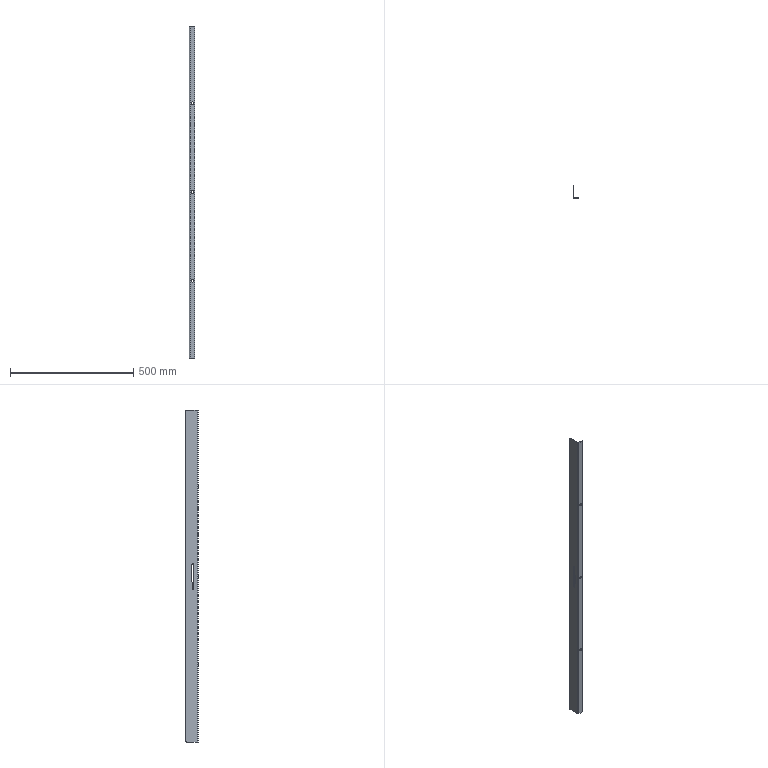Component | SolidWorks | RearRightSidePlateAssembly-1_RearRightSidePanelVerticalRib1-1 | 1 solid | 29 faces | box 24 x 50 x 1345 mm | volume 188474 mm3 | plane 18 | cylinder 11 | commonest cylinder face diameters 10 x6 6 x3 8 x1 4 x1 | material Plain Carbon Steel
STEP:
#1=CARTESIAN_POINT('',(78.003,47.699,67.145));
#2=VERTEX_POINT('',#1);
#3=CARTESIAN_POINT('',(78.003,47.699,67.539));
#4=VERTEX_POINT('',#3);
#5=CARTESIAN_POINT('',(78.003,47.699,67.342));
#6=DIRECTION('',(-0.,1.,0.));
#7=DIRECTION('',(0.,0.,1.));
#8=AXIS2_PLACEMENT_3D('',#5,#6,#7);
#9=CIRCLE('',#8,0.1969);
#10=EDGE_CURVE('',#2,#4,#9,.T.);
#11=ORIENTED_EDGE('',*,*,#10,.F.);
#12=CARTESIAN_POINT('',(78.003,47.778,67.145));
#13=VERTEX_POINT('',#12);
#14=CARTESIAN_POINT('',(78.003,47.699,67.145));
#15=DIRECTION('',(-0.,1.,0.));
#16=VECTOR('',#15,39.37);
#17=LINE('',#14,#16);
#18=EDGE_CURVE('',#2,#13,#17,.T.);
#19=ORIENTED_EDGE('',*,*,#18,.T.);
#20=CARTESIAN_POINT('',(78.003,47.778,67.539));
#21=VERTEX_POINT('',#20);
#22=CARTESIAN_POINT('',(78.003,47.778,67.342));
#23=DIRECTION('',(-0.,1.,0.));
#24=DIRECTION('',(0.,0.,1.));
#25=AXIS2_PLACEMENT_3D('',#22,#23,#24);
#26=CIRCLE('',#25,0.1969);
#27=EDGE_CURVE('',#13,#21,#26,.T.);
#28=ORIENTED_EDGE('',*,*,#27,.T.);
#29=CARTESIAN_POINT('',(78.003,47.699,67.539));
#30=DIRECTION('',(-0.,1.,0.));
#31=VECTOR('',#30,39.37);
#32=LINE('',#29,#31);
#33=EDGE_CURVE('',#4,#21,#32,.T.);
#34=ORIENTED_EDGE('',*,*,#33,.F.);
#35=EDGE_LOOP('',(#11,#19,#28,#34));
#36=FACE_OUTER_BOUND('',#35,.T.);
#37=CARTESIAN_POINT('',(78.003,47.699,67.342));
#38=DIRECTION('',(-0.,1.,0.));
#39=DIRECTION('',(0.,0.,1.));
#40=AXIS2_PLACEMENT_3D('',#37,#38,#39);
#41=CYLINDRICAL_SURFACE('',#40,0.1969);
#42=ADVANCED_FACE('',(#36),#41,.F.);
#43=CARTESIAN_POINT('',(78.003,47.699,38.798));
#44=VERTEX_POINT('',#43);
#45=CARTESIAN_POINT('',(78.003,47.699,39.192));
#46=VERTEX_POINT('',#45);
#47=CARTESIAN_POINT('',(78.003,47.699,38.995));
#48=DIRECTION('',(-0.,1.,0.));
#49=DIRECTION('',(0.,0.,1.));
#50=AXIS2_PLACEMENT_3D('',#47,#48,#49);
#51=CIRCLE('',#50,0.1969);
#52=EDGE_CURVE('',#44,#46,#51,.T.);
#53=ORIENTED_EDGE('',*,*,#52,.F.);
#54=CARTESIAN_POINT('',(78.003,47.778,38.798));
#55=VERTEX_POINT('',#54);
#56=CARTESIAN_POINT('',(78.003,47.699,38.798));
#57=DIRECTION('',(-0.,1.,0.));
#58=VECTOR('',#57,39.37);
#59=LINE('',#56,#58);
#60=EDGE_CURVE('',#44,#55,#59,.T.);
#61=ORIENTED_EDGE('',*,*,#60,.T.);
#62=CARTESIAN_POINT('',(78.003,47.778,39.192));
#63=VERTEX_POINT('',#62);
#64=CARTESIAN_POINT('',(78.003,47.778,38.995));
#65=DIRECTION('',(-0.,1.,0.));
#66=DIRECTION('',(0.,0.,1.));
#67=AXIS2_PLACEMENT_3D('',#64,#65,#66);
#68=CIRCLE('',#67,0.1969);
#69=EDGE_CURVE('',#55,#63,#68,.T.);
#70=ORIENTED_EDGE('',*,*,#69,.T.);
#71=CARTESIAN_POINT('',(78.003,47.699,39.192));
#72=DIRECTION('',(-0.,1.,0.));
#73=VECTOR('',#72,39.37);
#74=LINE('',#71,#73);
#75=EDGE_CURVE('',#46,#63,#74,.T.);
#76=ORIENTED_EDGE('',*,*,#75,.F.);
#77=EDGE_LOOP('',(#53,#61,#70,#76));
#78=FACE_OUTER_BOUND('',#77,.T.);
#79=CARTESIAN_POINT('',(78.003,47.699,38.995));
#80=DIRECTION('',(-0.,1.,0.));
#81=DIRECTION('',(0.,0.,1.));
#82=AXIS2_PLACEMENT_3D('',#79,#80,#81);
#83=CYLINDRICAL_SURFACE('',#82,0.1969);
#84=ADVANCED_FACE('',(#78),#83,.F.);
#85=CARTESIAN_POINT('',(78.003,47.699,52.972));
#86=VERTEX_POINT('',#85);
#87=CARTESIAN_POINT('',(78.003,47.699,53.365));
#88=VERTEX_POINT('',#87);
#89=CARTESIAN_POINT('',(78.003,47.699,53.168));
#90=DIRECTION('',(-0.,1.,0.));
#91=DIRECTION('',(0.,0.,1.));
#92=AXIS2_PLACEMENT_3D('',#89,#90,#91);
#93=CIRCLE('',#92,0.1969);
#94=EDGE_CURVE('',#86,#88,#93,.T.);
#95=ORIENTED_EDGE('',*,*,#94,.F.);
#96=CARTESIAN_POINT('',(78.003,47.778,52.972));
#97=VERTEX_POINT('',#96);
#98=CARTESIAN_POINT('',(78.003,47.699,52.972));
#99=DIRECTION('',(-0.,1.,0.));
#100=VECTOR('',#99,39.37);
#101=LINE('',#98,#100);
#102=EDGE_CURVE('',#86,#97,#101,.T.);
#103=ORIENTED_EDGE('',*,*,#102,.T.);
#104=CARTESIAN_POINT('',(78.003,47.778,53.365));
#105=VERTEX_POINT('',#104);
#106=CARTESIAN_POINT('',(78.003,47.778,53.168));
#107=DIRECTION('',(-0.,1.,0.));
#108=DIRECTION('',(0.,0.,1.));
#109=AXIS2_PLACEMENT_3D('',#106,#107,#108);
#110=CIRCLE('',#109,0.1969);
#111=EDGE_CURVE('',#97,#105,#110,.T.);
#112=ORIENTED_EDGE('',*,*,#111,.T.);
#113=CARTESIAN_POINT('',(78.003,47.699,53.365));
#114=DIRECTION('',(-0.,1.,0.));
#115=VECTOR('',#114,39.37);
#116=LINE('',#113,#115);
#117=EDGE_CURVE('',#88,#105,#116,.T.);
#118=ORIENTED_EDGE('',*,*,#117,.F.);
#119=EDGE_LOOP('',(#95,#103,#112,#118));
#120=FACE_OUTER_BOUND('',#119,.T.);
#121=CARTESIAN_POINT('',(78.003,47.699,53.168));
#122=DIRECTION('',(-0.,1.,0.));
#123=DIRECTION('',(0.,0.,1.));
#124=AXIS2_PLACEMENT_3D('',#121,#122,#123);
#125=CYLINDRICAL_SURFACE('',#124,0.1969);
#126=ADVANCED_FACE('',(#120),#125,.F.);
#127=CARTESIAN_POINT('',(77.531,48.565,50.983));
#128=VERTEX_POINT('',#127);
#129=CARTESIAN_POINT('',(77.531,48.447,51.102));
#130=VERTEX_POINT('',#129);
#131=CARTESIAN_POINT('',(77.531,48.565,51.102));
#132=DIRECTION('',(-1.,-0.,0.));
#133=DIRECTION('',(0.,0.,-1.));
#134=AXIS2_PLACEMENT_3D('',#131,#132,#133);
#135=CIRCLE('',#134,0.1181);
#136=EDGE_CURVE('',#128,#130,#135,.T.);
#137=ORIENTED_EDGE('',*,*,#136,.F.);
#138=CARTESIAN_POINT('',(77.452,48.565,50.983));
#139=VERTEX_POINT('',#138);
#140=CARTESIAN_POINT('',(77.531,48.565,50.983));
#141=DIRECTION('',(-1.,-0.,0.));
#142=VECTOR('',#141,39.37);
#143=LINE('',#140,#142);
#144=EDGE_CURVE('',#128,#139,#143,.T.);
#145=ORIENTED_EDGE('',*,*,#144,.T.);
#146=CARTESIAN_POINT('',(77.452,48.447,51.102));
#147=VERTEX_POINT('',#146);
#148=CARTESIAN_POINT('',(77.452,48.565,51.102));
#149=DIRECTION('',(-1.,-0.,0.));
#150=DIRECTION('',(0.,0.,-1.));
#151=AXIS2_PLACEMENT_3D('',#148,#149,#150);
#152=CIRCLE('',#151,0.1181);
#153=EDGE_CURVE('',#139,#147,#152,.T.);
#154=ORIENTED_EDGE('',*,*,#153,.T.);
#155=CARTESIAN_POINT('',(77.531,48.447,51.102));
#156=DIRECTION('',(-1.,-0.,0.));
#157=VECTOR('',#156,39.37);
#158=LINE('',#155,#157);
#159=EDGE_CURVE('',#130,#147,#158,.T.);
#160=ORIENTED_EDGE('',*,*,#159,.F.);
#161=EDGE_LOOP('',(#137,#145,#154,#160));
#162=FACE_OUTER_BOUND('',#161,.T.);
#163=CARTESIAN_POINT('',(77.531,48.565,51.102));
#164=DIRECTION('',(-1.,-0.,0.));
#165=DIRECTION('',(0.,0.,-1.));
#166=AXIS2_PLACEMENT_3D('',#163,#164,#165);
#167=CYLINDRICAL_SURFACE('',#166,0.1181);
#168=ADVANCED_FACE('',(#162),#167,.F.);
#169=CARTESIAN_POINT('',(77.452,48.683,51.102));
#170=VERTEX_POINT('',#169);
#171=CARTESIAN_POINT('',(77.452,48.565,51.102));
#172=DIRECTION('',(-1.,-0.,0.));
#173=DIRECTION('',(0.,0.,-1.));
#174=AXIS2_PLACEMENT_3D('',#171,#172,#173);
#175=CIRCLE('',#174,0.1181);
#176=EDGE_CURVE('',#170,#139,#175,.T.);
#177=ORIENTED_EDGE('',*,*,#176,.F.);
#178=CARTESIAN_POINT('',(77.452,48.683,55.039));
#179=VERTEX_POINT('',#178);
#180=CARTESIAN_POINT('',(77.452,48.683,51.102));
#181=DIRECTION('',(-0.,-0.,-1.));
#182=VECTOR('',#181,39.37);
#183=LINE('',#180,#182);
#184=EDGE_CURVE('',#179,#170,#183,.T.);
#185=ORIENTED_EDGE('',*,*,#184,.F.);
#186=CARTESIAN_POINT('',(77.452,48.447,55.039));
#187=VERTEX_POINT('',#186);
#188=CARTESIAN_POINT('',(77.452,48.565,55.039));
#189=DIRECTION('',(-1.,-0.,0.));
#190=DIRECTION('',(0.,0.,-1.));
#191=AXIS2_PLACEMENT_3D('',#188,#189,#190);
#192=CIRCLE('',#191,0.1181);
#193=EDGE_CURVE('',#187,#179,#192,.T.);
#194=ORIENTED_EDGE('',*,*,#193,.F.);
#195=CARTESIAN_POINT('',(77.452,48.447,51.102));
#196=DIRECTION('',(0.,0.,1.));
#197=VECTOR('',#196,39.37);
#198=LINE('',#195,#197);
#199=EDGE_CURVE('',#147,#187,#198,.T.);
#200=ORIENTED_EDGE('',*,*,#199,.F.);
#201=ORIENTED_EDGE('',*,*,#153,.F.);
#202=EDGE_LOOP('',(#177,#185,#194,#200,#201));
#203=FACE_BOUND('',#202,.T.);
#204=CARTESIAN_POINT('',(77.452,49.667,26.759));
#205=VERTEX_POINT('',#204);
#206=CARTESIAN_POINT('',(77.452,49.667,79.578));
#207=VERTEX_POINT('',#206);
#208=CARTESIAN_POINT('',(77.452,49.667,26.692));
#209=DIRECTION('',(0.,-0.,1.));
#210=VECTOR('',#209,39.37);
#211=LINE('',#208,#210);
#212=EDGE_CURVE('',#205,#207,#211,.T.);
#213=ORIENTED_EDGE('',*,*,#212,.F.);
#214=CARTESIAN_POINT('',(77.452,49.581,26.759));
#215=VERTEX_POINT('',#214);
#216=CARTESIAN_POINT('',(77.452,49.667,26.759));
#217=DIRECTION('',(0.,-1.,-0.));
#218=VECTOR('',#217,39.37);
#219=LINE('',#216,#218);
#220=EDGE_CURVE('',#205,#215,#219,.T.);
#221=ORIENTED_EDGE('',*,*,#220,.T.);
#222=CARTESIAN_POINT('',(77.452,49.581,26.692));
#223=VERTEX_POINT('',#222);
#224=CARTESIAN_POINT('',(77.452,49.581,26.692));
#225=DIRECTION('',(-0.,0.,-1.));
#226=VECTOR('',#225,39.37);
#227=LINE('',#224,#226);
#228=EDGE_CURVE('',#215,#223,#227,.T.);
#229=ORIENTED_EDGE('',*,*,#228,.T.);
#230=CARTESIAN_POINT('',(77.452,47.856,26.692));
#231=VERTEX_POINT('',#230);
#232=CARTESIAN_POINT('',(77.452,49.667,26.692));
#233=DIRECTION('',(0.,-1.,-0.));
#234=VECTOR('',#233,39.37);
#235=LINE('',#232,#234);
#236=EDGE_CURVE('',#223,#231,#235,.T.);
#237=ORIENTED_EDGE('',*,*,#236,.T.);
#238=CARTESIAN_POINT('',(77.452,47.856,79.645));
#239=VERTEX_POINT('',#238);
#240=CARTESIAN_POINT('',(77.452,47.856,26.692));
#241=DIRECTION('',(0.,-0.,1.));
#242=VECTOR('',#241,39.37);
#243=LINE('',#240,#242);
#244=EDGE_CURVE('',#231,#239,#243,.T.);
#245=ORIENTED_EDGE('',*,*,#244,.T.);
#246=CARTESIAN_POINT('',(77.452,49.581,79.645));
#247=VERTEX_POINT('',#246);
#248=CARTESIAN_POINT('',(77.452,49.667,79.645));
#249=DIRECTION('',(0.,-1.,-0.));
#250=VECTOR('',#249,39.37);
#251=LINE('',#248,#250);
#252=EDGE_CURVE('',#247,#239,#251,.T.);
#253=ORIENTED_EDGE('',*,*,#252,.F.);
#254=CARTESIAN_POINT('',(77.452,49.581,79.578));
#255=VERTEX_POINT('',#254);
#256=CARTESIAN_POINT('',(77.452,49.581,26.692));
#257=DIRECTION('',(-0.,0.,-1.));
#258=VECTOR('',#257,39.37);
#259=LINE('',#256,#258);
#260=EDGE_CURVE('',#247,#255,#259,.T.);
#261=ORIENTED_EDGE('',*,*,#260,.T.);
#262=CARTESIAN_POINT('',(77.452,49.667,79.578));
#263=DIRECTION('',(-0.,1.,0.));
#264=VECTOR('',#263,39.37);
#265=LINE('',#262,#264);
#266=EDGE_CURVE('',#255,#207,#265,.T.);
#267=ORIENTED_EDGE('',*,*,#266,.T.);
#268=EDGE_LOOP('',(#213,#221,#229,#237,#245,#253,#261,#267));
#269=FACE_OUTER_BOUND('',#268,.T.);
#270=CARTESIAN_POINT('',(77.452,49.667,26.692));
#271=DIRECTION('',(-1.,-0.,0.));
#272=DIRECTION('',(-0.,0.,-1.));
#273=AXIS2_PLACEMENT_3D('',#270,#271,#272);
#274=PLANE('',#273);
#275=ADVANCED_FACE('',(#203,#269),#274,.T.);
#276=CARTESIAN_POINT('',(77.61,47.699,26.692));
#277=VERTEX_POINT('',#276);
#278=CARTESIAN_POINT('',(77.61,47.778,26.692));
#279=VERTEX_POINT('',#278);
#280=CARTESIAN_POINT('',(77.61,47.699,26.692));
#281=DIRECTION('',(-0.,1.,0.));
#282=VECTOR('',#281,39.37);
#283=LINE('',#280,#282);
#284=EDGE_CURVE('',#277,#279,#283,.T.);
#285=ORIENTED_EDGE('',*,*,#284,.F.);
#286=CARTESIAN_POINT('',(77.61,47.856,26.692));
#287=DIRECTION('',(0.,-0.,1.));
#288=DIRECTION('',(1.,0.,0.));
#289=AXIS2_PLACEMENT_3D('',#286,#287,#288);
#290=CIRCLE('',#289,0.1575);
#291=EDGE_CURVE('',#231,#277,#290,.T.);
#292=ORIENTED_EDGE('',*,*,#291,.F.);
#293=CARTESIAN_POINT('',(77.531,47.856,26.692));
#294=VERTEX_POINT('',#293);
#295=CARTESIAN_POINT('',(77.531,47.856,26.692));
#296=DIRECTION('',(-1.,-0.,0.));
#297=VECTOR('',#296,39.37);
#298=LINE('',#295,#297);
#299=EDGE_CURVE('',#294,#231,#298,.T.);
#300=ORIENTED_EDGE('',*,*,#299,.F.);
#301=CARTESIAN_POINT('',(77.61,47.856,26.692));
#302=DIRECTION('',(0.,-0.,1.));
#303=DIRECTION('',(1.,0.,0.));
#304=AXIS2_PLACEMENT_3D('',#301,#302,#303);
#305=CIRCLE('',#304,0.07874);
#306=EDGE_CURVE('',#294,#279,#305,.T.);
#307=ORIENTED_EDGE('',*,*,#306,.T.);
#308=EDGE_LOOP('',(#285,#292,#300,#307));
#309=FACE_OUTER_BOUND('',#308,.T.);
#310=CARTESIAN_POINT('',(77.61,47.699,26.692));
#311=DIRECTION('',(-0.,0.,-1.));
#312=DIRECTION('',(1.,0.,-0.));
#313=AXIS2_PLACEMENT_3D('',#310,#311,#312);
#314=PLANE('',#313);
#315=ADVANCED_FACE('',(#309),#314,.T.);
#316=CARTESIAN_POINT('',(78.397,47.699,26.692));
#317=VERTEX_POINT('',#316);
#318=CARTESIAN_POINT('',(77.452,47.699,26.692));
#319=DIRECTION('',(1.,0.,-0.));
#320=VECTOR('',#319,39.37);
#321=LINE('',#318,#320);
#322=EDGE_CURVE('',#277,#317,#321,.T.);
#323=ORIENTED_EDGE('',*,*,#322,.F.);
#324=ORIENTED_EDGE('',*,*,#284,.T.);
#325=CARTESIAN_POINT('',(78.397,47.778,26.692));
#326=VERTEX_POINT('',#325);
#327=CARTESIAN_POINT('',(77.452,47.778,26.692));
#328=DIRECTION('',(1.,0.,-0.));
#329=VECTOR('',#328,39.37);
#330=LINE('',#327,#329);
#331=EDGE_CURVE('',#279,#326,#330,.T.);
#332=ORIENTED_EDGE('',*,*,#331,.T.);
#333=CARTESIAN_POINT('',(78.397,47.699,26.692));
#334=DIRECTION('',(-0.,1.,0.));
#335=VECTOR('',#334,39.37);
#336=LINE('',#333,#335);
#337=EDGE_CURVE('',#317,#326,#336,.T.);
#338=ORIENTED_EDGE('',*,*,#337,.F.);
#339=EDGE_LOOP('',(#323,#324,#332,#338));
#340=FACE_OUTER_BOUND('',#339,.T.);
#341=CARTESIAN_POINT('',(77.531,47.856,26.692));
#342=DIRECTION('',(-0.,0.,-1.));
#343=DIRECTION('',(1.,0.,-0.));
#344=AXIS2_PLACEMENT_3D('',#341,#342,#343);
#345=PLANE('',#344);
#346=ADVANCED_FACE('',(#340),#345,.T.);
#347=CARTESIAN_POINT('',(77.531,47.856,79.645));
#348=VERTEX_POINT('',#347);
#349=CARTESIAN_POINT('',(77.452,47.856,79.645));
#350=DIRECTION('',(1.,0.,-0.));
#351=VECTOR('',#350,39.37);
#352=LINE('',#349,#351);
#353=EDGE_CURVE('',#239,#348,#352,.T.);
#354=ORIENTED_EDGE('',*,*,#353,.F.);
#355=CARTESIAN_POINT('',(77.61,47.699,79.645));
#356=VERTEX_POINT('',#355);
#357=CARTESIAN_POINT('',(77.61,47.856,79.645));
#358=DIRECTION('',(0.,-0.,1.));
#359=DIRECTION('',(1.,0.,0.));
#360=AXIS2_PLACEMENT_3D('',#357,#358,#359);
#361=CIRCLE('',#360,0.1575);
#362=EDGE_CURVE('',#239,#356,#361,.T.);
#363=ORIENTED_EDGE('',*,*,#362,.T.);
#364=CARTESIAN_POINT('',(77.61,47.778,79.645));
#365=VERTEX_POINT('',#364);
#366=CARTESIAN_POINT('',(77.61,47.778,79.645));
#367=DIRECTION('',(0.,-1.,-0.));
#368=VECTOR('',#367,39.37);
#369=LINE('',#366,#368);
#370=EDGE_CURVE('',#365,#356,#369,.T.);
#371=ORIENTED_EDGE('',*,*,#370,.F.);
#372=CARTESIAN_POINT('',(77.61,47.856,79.645));
#373=DIRECTION('',(0.,-0.,1.));
#374=DIRECTION('',(1.,0.,0.));
#375=AXIS2_PLACEMENT_3D('',#372,#373,#374);
#376=CIRCLE('',#375,0.07874);
#377=EDGE_CURVE('',#348,#365,#376,.T.);
#378=ORIENTED_EDGE('',*,*,#377,.F.);
#379=EDGE_LOOP('',(#354,#363,#371,#378));
#380=FACE_OUTER_BOUND('',#379,.T.);
#381=CARTESIAN_POINT('',(77.452,47.856,79.645));
#382=DIRECTION('',(0.,-0.,1.));
#383=DIRECTION('',(-1.,-0.,0.));
#384=AXIS2_PLACEMENT_3D('',#381,#382,#383);
#385=PLANE('',#384);
#386=ADVANCED_FACE('',(#380),#385,.T.);
#387=CARTESIAN_POINT('',(77.531,49.581,79.645));
#388=VERTEX_POINT('',#387);
#389=CARTESIAN_POINT('',(77.61,49.581,79.645));
#390=DIRECTION('',(1.,0.,-0.));
#391=VECTOR('',#390,39.37);
#392=LINE('',#389,#391);
#393=EDGE_CURVE('',#247,#388,#392,.T.);
#394=ORIENTED_EDGE('',*,*,#393,.F.);
#395=ORIENTED_EDGE('',*,*,#252,.T.);
#396=ORIENTED_EDGE('',*,*,#353,.T.);
#397=CARTESIAN_POINT('',(77.531,49.667,79.645));
#398=DIRECTION('',(0.,-1.,-0.));
#399=VECTOR('',#398,39.37);
#400=LINE('',#397,#399);
#401=EDGE_CURVE('',#388,#348,#400,.T.);
#402=ORIENTED_EDGE('',*,*,#401,.F.);
#403=EDGE_LOOP('',(#394,#395,#396,#402));
#404=FACE_OUTER_BOUND('',#403,.T.);
#405=CARTESIAN_POINT('',(77.61,47.778,79.645));
#406=DIRECTION('',(0.,-0.,1.));
#407=DIRECTION('',(-1.,-0.,0.));
#408=AXIS2_PLACEMENT_3D('',#405,#406,#407);
#409=PLANE('',#408);
#410=ADVANCED_FACE('',(#404),#409,.T.);
#411=CARTESIAN_POINT('',(78.003,47.778,67.342));
#412=DIRECTION('',(-0.,1.,0.));
#413=DIRECTION('',(0.,0.,1.));
#414=AXIS2_PLACEMENT_3D('',#411,#412,#413);
#415=CIRCLE('',#414,0.1969);
#416=EDGE_CURVE('',#21,#13,#415,.T.);
#417=ORIENTED_EDGE('',*,*,#416,.F.);
#418=ORIENTED_EDGE('',*,*,#27,.F.);
#419=EDGE_LOOP('',(#417,#418));
#420=FACE_BOUND('',#419,.T.);
#421=CARTESIAN_POINT('',(78.003,47.778,38.995));
#422=DIRECTION('',(-0.,1.,0.));
#423=DIRECTION('',(0.,0.,1.));
#424=AXIS2_PLACEMENT_3D('',#421,#422,#423);
#425=CIRCLE('',#424,0.1969);
#426=EDGE_CURVE('',#63,#55,#425,.T.);
#427=ORIENTED_EDGE('',*,*,#426,.F.);
#428=ORIENTED_EDGE('',*,*,#69,.F.);
#429=EDGE_LOOP('',(#427,#428));
#430=FACE_BOUND('',#429,.T.);
#431=CARTESIAN_POINT('',(78.003,47.778,53.168));
#432=DIRECTION('',(-0.,1.,0.));
#433=DIRECTION('',(0.,0.,1.));
#434=AXIS2_PLACEMENT_3D('',#431,#432,#433);
#435=CIRCLE('',#434,0.1969);
#436=EDGE_CURVE('',#105,#97,#435,.T.);
#437=ORIENTED_EDGE('',*,*,#436,.F.);
#438=ORIENTED_EDGE('',*,*,#111,.F.);
#439=EDGE_LOOP('',(#437,#438));
#440=FACE_BOUND('',#439,.T.);
#441=CARTESIAN_POINT('',(78.397,47.778,79.645));
#442=VERTEX_POINT('',#441);
#443=CARTESIAN_POINT('',(77.452,47.778,79.645));
#444=DIRECTION('',(1.,0.,-0.));
#445=VECTOR('',#444,39.37);
#446=LINE('',#443,#445);
#447=EDGE_CURVE('',#365,#442,#446,.T.);
#448=ORIENTED_EDGE('',*,*,#447,.T.);
#449=CARTESIAN_POINT('',(78.397,47.778,26.692));
#450=DIRECTION('',(0.,-0.,1.));
#451=VECTOR('',#450,39.37);
#452=LINE('',#449,#451);
#453=EDGE_CURVE('',#326,#442,#452,.T.);
#454=ORIENTED_EDGE('',*,*,#453,.F.);
#455=ORIENTED_EDGE('',*,*,#331,.F.);
#456=CARTESIAN_POINT('',(77.61,47.778,26.692));
#457=DIRECTION('',(0.,-0.,1.));
#458=VECTOR('',#457,39.37);
#459=LINE('',#456,#458);
#460=EDGE_CURVE('',#279,#365,#459,.T.);
#461=ORIENTED_EDGE('',*,*,#460,.T.);
#462=EDGE_LOOP('',(#448,#454,#455,#461));
#463=FACE_OUTER_BOUND('',#462,.T.);
#464=CARTESIAN_POINT('',(77.452,47.778,26.692));
#465=DIRECTION('',(0.,-1.,-0.));
#466=DIRECTION('',(-0.,0.,-1.));
#467=AXIS2_PLACEMENT_3D('',#464,#465,#466);
#468=PLANE('',#467);
#469=ADVANCED_FACE('',(#420,#430,#440,#463),#468,.F.);
#470=CARTESIAN_POINT('',(78.397,47.699,79.645));
#471=VERTEX_POINT('',#470);
#472=CARTESIAN_POINT('',(78.397,47.699,79.645));
#473=DIRECTION('',(-0.,1.,0.));
#474=VECTOR('',#473,39.37);
#475=LINE('',#472,#474);
#476=EDGE_CURVE('',#471,#442,#475,.T.);
#477=ORIENTED_EDGE('',*,*,#476,.F.);
#478=CARTESIAN_POINT('',(78.397,47.699,26.692));
#479=DIRECTION('',(0.,-0.,1.));
#480=VECTOR('',#479,39.37);
#481=LINE('',#478,#480);
#482=EDGE_CURVE('',#317,#471,#481,.T.);
#483=ORIENTED_EDGE('',*,*,#482,.F.);
#484=ORIENTED_EDGE('',*,*,#337,.T.);
#485=ORIENTED_EDGE('',*,*,#453,.T.);
#486=EDGE_LOOP('',(#477,#483,#484,#485));
#487=FACE_OUTER_BOUND('',#486,.T.);
#488=CARTESIAN_POINT('',(78.397,47.699,26.692));
#489=DIRECTION('',(1.,0.,-0.));
#490=DIRECTION('',(0.,-0.,1.));
#491=AXIS2_PLACEMENT_3D('',#488,#489,#490);
#492=PLANE('',#491);
#493=ADVANCED_FACE('',(#487),#492,.T.);
#494=CARTESIAN_POINT('',(78.003,47.699,67.342));
#495=DIRECTION('',(-0.,1.,0.));
#496=DIRECTION('',(0.,0.,1.));
#497=AXIS2_PLACEMENT_3D('',#494,#495,#496);
#498=CIRCLE('',#497,0.1969);
#499=EDGE_CURVE('',#4,#2,#498,.T.);
#500=ORIENTED_EDGE('',*,*,#499,.T.);
#501=ORIENTED_EDGE('',*,*,#10,.T.);
#502=EDGE_LOOP('',(#500,#501));
#503=FACE_BOUND('',#502,.T.);
#504=CARTESIAN_POINT('',(78.003,47.699,38.995));
#505=DIRECTION('',(-0.,1.,0.));
#506=DIRECTION('',(0.,0.,1.));
#507=AXIS2_PLACEMENT_3D('',#504,#505,#506);
#508=CIRCLE('',#507,0.1969);
#509=EDGE_CURVE('',#46,#44,#508,.T.);
#510=ORIENTED_EDGE('',*,*,#509,.T.);
#511=ORIENTED_EDGE('',*,*,#52,.T.);
#512=EDGE_LOOP('',(#510,#511));
#513=FACE_BOUND('',#512,.T.);
#514=CARTESIAN_POINT('',(78.003,47.699,53.168));
#515=DIRECTION('',(-0.,1.,0.));
#516=DIRECTION('',(0.,0.,1.));
#517=AXIS2_PLACEMENT_3D('',#514,#515,#516);
#518=CIRCLE('',#517,0.1969);
#519=EDGE_CURVE('',#88,#86,#518,.T.);
#520=ORIENTED_EDGE('',*,*,#519,.T.);
#521=ORIENTED_EDGE('',*,*,#94,.T.);
#522=EDGE_LOOP('',(#520,#521));
#523=FACE_BOUND('',#522,.T.);
#524=CARTESIAN_POINT('',(77.452,47.699,79.645));
#525=DIRECTION('',(1.,0.,-0.));
#526=VECTOR('',#525,39.37);
#527=LINE('',#524,#526);
#528=EDGE_CURVE('',#356,#471,#527,.T.);
#529=ORIENTED_EDGE('',*,*,#528,.F.);
#530=CARTESIAN_POINT('',(77.61,47.699,26.692));
#531=DIRECTION('',(0.,-0.,1.));
#532=VECTOR('',#531,39.37);
#533=LINE('',#530,#532);
#534=EDGE_CURVE('',#277,#356,#533,.T.);
#535=ORIENTED_EDGE('',*,*,#534,.F.);
#536=ORIENTED_EDGE('',*,*,#322,.T.);
#537=ORIENTED_EDGE('',*,*,#482,.T.);
#538=EDGE_LOOP('',(#529,#535,#536,#537));
#539=FACE_OUTER_BOUND('',#538,.T.);
#540=CARTESIAN_POINT('',(77.452,47.699,26.692));
#541=DIRECTION('',(0.,-1.,-0.));
#542=DIRECTION('',(-0.,0.,-1.));
#543=AXIS2_PLACEMENT_3D('',#540,#541,#542);
#544=PLANE('',#543);
#545=ADVANCED_FACE('',(#503,#513,#523,#539),#544,.T.);
#546=ORIENTED_EDGE('',*,*,#362,.F.);
#547=ORIENTED_EDGE('',*,*,#244,.F.);
#548=ORIENTED_EDGE('',*,*,#291,.T.);
#549=ORIENTED_EDGE('',*,*,#534,.T.);
#550=EDGE_LOOP('',(#546,#547,#548,#549));
#551=FACE_OUTER_BOUND('',#550,.T.);
#552=CARTESIAN_POINT('',(77.61,47.856,26.692));
#553=DIRECTION('',(0.,-0.,1.));
#554=DIRECTION('',(-1.,0.,0.));
#555=AXIS2_PLACEMENT_3D('',#552,#553,#554);
#556=CYLINDRICAL_SURFACE('',#555,0.1575);
#557=ADVANCED_FACE('',(#551),#556,.T.);
#558=CARTESIAN_POINT('',(77.531,49.667,26.759));
#559=VERTEX_POINT('',#558);
#560=CARTESIAN_POINT('',(77.531,49.667,26.759));
#561=DIRECTION('',(1.,0.,-0.));
#562=VECTOR('',#561,39.37);
#563=LINE('',#560,#562);
#564=EDGE_CURVE('',#205,#559,#563,.T.);
#565=ORIENTED_EDGE('',*,*,#564,.F.);
#566=ORIENTED_EDGE('',*,*,#212,.T.);
#567=CARTESIAN_POINT('',(77.531,49.667,79.578));
#568=VERTEX_POINT('',#567);
#569=CARTESIAN_POINT('',(77.531,49.667,79.578));
#570=DIRECTION('',(-1.,-0.,0.));
#571=VECTOR('',#570,39.37);
#572=LINE('',#569,#571);
#573=EDGE_CURVE('',#568,#207,#572,.T.);
#574=ORIENTED_EDGE('',*,*,#573,.F.);
#575=CARTESIAN_POINT('',(77.531,49.667,26.692));
#576=DIRECTION('',(0.,-0.,1.));
#577=VECTOR('',#576,39.37);
#578=LINE('',#575,#577);
#579=EDGE_CURVE('',#559,#568,#578,.T.);
#580=ORIENTED_EDGE('',*,*,#579,.F.);
#581=EDGE_LOOP('',(#565,#566,#574,#580));
#582=FACE_OUTER_BOUND('',#581,.T.);
#583=CARTESIAN_POINT('',(77.531,49.667,26.692));
#584=DIRECTION('',(-0.,1.,0.));
#585=DIRECTION('',(0.,-0.,1.));
#586=AXIS2_PLACEMENT_3D('',#583,#584,#585);
#587=PLANE('',#586);
#588=ADVANCED_FACE('',(#582),#587,.T.);
#589=CARTESIAN_POINT('',(77.531,48.683,55.039));
#590=VERTEX_POINT('',#589);
#591=CARTESIAN_POINT('',(77.531,48.683,51.102));
#592=VERTEX_POINT('',#591);
#593=CARTESIAN_POINT('',(77.531,48.683,51.102));
#594=DIRECTION('',(-0.,-0.,-1.));
#595=VECTOR('',#594,39.37);
#596=LINE('',#593,#595);
#597=EDGE_CURVE('',#590,#592,#596,.T.);
#598=ORIENTED_EDGE('',*,*,#597,.T.);
#599=CARTESIAN_POINT('',(77.531,48.565,51.102));
#600=DIRECTION('',(-1.,-0.,0.));
#601=DIRECTION('',(0.,0.,-1.));
#602=AXIS2_PLACEMENT_3D('',#599,#600,#601);
#603=CIRCLE('',#602,0.1181);
#604=EDGE_CURVE('',#592,#128,#603,.T.);
#605=ORIENTED_EDGE('',*,*,#604,.T.);
#606=ORIENTED_EDGE('',*,*,#136,.T.);
#607=CARTESIAN_POINT('',(77.531,48.447,55.039));
#608=VERTEX_POINT('',#607);
#609=CARTESIAN_POINT('',(77.531,48.447,51.102));
#610=DIRECTION('',(0.,0.,1.));
#611=VECTOR('',#610,39.37);
#612=LINE('',#609,#611);
#613=EDGE_CURVE('',#130,#608,#612,.T.);
#614=ORIENTED_EDGE('',*,*,#613,.T.);
#615=CARTESIAN_POINT('',(77.531,48.565,55.039));
#616=DIRECTION('',(-1.,-0.,0.));
#617=DIRECTION('',(0.,0.,-1.));
#618=AXIS2_PLACEMENT_3D('',#615,#616,#617);
#619=CIRCLE('',#618,0.1181);
#620=EDGE_CURVE('',#608,#590,#619,.T.);
#621=ORIENTED_EDGE('',*,*,#620,.T.);
#622=EDGE_LOOP('',(#598,#605,#606,#614,#621));
#623=FACE_BOUND('',#622,.T.);
#624=CARTESIAN_POINT('',(77.531,49.581,26.692));
#625=VERTEX_POINT('',#624);
#626=CARTESIAN_POINT('',(77.531,49.581,26.759));
#627=VERTEX_POINT('',#626);
#628=CARTESIAN_POINT('',(77.531,49.581,26.692));
#629=DIRECTION('',(0.,-0.,1.));
#630=VECTOR('',#629,39.37);
#631=LINE('',#628,#630);
#632=EDGE_CURVE('',#625,#627,#631,.T.);
#633=ORIENTED_EDGE('',*,*,#632,.T.);
#634=CARTESIAN_POINT('',(77.531,49.667,26.759));
#635=DIRECTION('',(-0.,1.,0.));
#636=VECTOR('',#635,39.37);
#637=LINE('',#634,#636);
#638=EDGE_CURVE('',#627,#559,#637,.T.);
#639=ORIENTED_EDGE('',*,*,#638,.T.);
#640=ORIENTED_EDGE('',*,*,#579,.T.);
#641=CARTESIAN_POINT('',(77.531,49.581,79.578));
#642=VERTEX_POINT('',#641);
#643=CARTESIAN_POINT('',(77.531,49.667,79.578));
#644=DIRECTION('',(0.,-1.,-0.));
#645=VECTOR('',#644,39.37);
#646=LINE('',#643,#645);
#647=EDGE_CURVE('',#568,#642,#646,.T.);
#648=ORIENTED_EDGE('',*,*,#647,.T.);
#649=CARTESIAN_POINT('',(77.531,49.581,26.692));
#650=DIRECTION('',(0.,-0.,1.));
#651=VECTOR('',#650,39.37);
#652=LINE('',#649,#651);
#653=EDGE_CURVE('',#642,#388,#652,.T.);
#654=ORIENTED_EDGE('',*,*,#653,.T.);
#655=ORIENTED_EDGE('',*,*,#401,.T.);
#656=CARTESIAN_POINT('',(77.531,47.856,26.692));
#657=DIRECTION('',(0.,-0.,1.));
#658=VECTOR('',#657,39.37);
#659=LINE('',#656,#658);
#660=EDGE_CURVE('',#294,#348,#659,.T.);
#661=ORIENTED_EDGE('',*,*,#660,.F.);
#662=CARTESIAN_POINT('',(77.531,49.667,26.692));
#663=DIRECTION('',(0.,-1.,-0.));
#664=VECTOR('',#663,39.37);
#665=LINE('',#662,#664);
#666=EDGE_CURVE('',#625,#294,#665,.T.);
#667=ORIENTED_EDGE('',*,*,#666,.F.);
#668=EDGE_LOOP('',(#633,#639,#640,#648,#654,#655,#661,#667));
#669=FACE_OUTER_BOUND('',#668,.T.);
#670=CARTESIAN_POINT('',(77.531,49.667,26.692));
#671=DIRECTION('',(-1.,-0.,0.));
#672=DIRECTION('',(-0.,0.,-1.));
#673=AXIS2_PLACEMENT_3D('',#670,#671,#672);
#674=PLANE('',#673);
#675=ADVANCED_FACE('',(#623,#669),#674,.F.);
#676=ORIENTED_EDGE('',*,*,#377,.T.);
#677=ORIENTED_EDGE('',*,*,#460,.F.);
#678=ORIENTED_EDGE('',*,*,#306,.F.);
#679=ORIENTED_EDGE('',*,*,#660,.T.);
#680=EDGE_LOOP('',(#676,#677,#678,#679));
#681=FACE_OUTER_BOUND('',#680,.T.);
#682=CARTESIAN_POINT('',(77.61,47.856,26.692));
#683=DIRECTION('',(0.,-0.,1.));
#684=DIRECTION('',(-1.,0.,0.));
#685=AXIS2_PLACEMENT_3D('',#682,#683,#684);
#686=CYLINDRICAL_SURFACE('',#685,0.07874);
#687=ADVANCED_FACE('',(#681),#686,.F.);
#688=CARTESIAN_POINT('',(77.61,49.581,26.692));
#689=DIRECTION('',(-1.,-0.,0.));
#690=VECTOR('',#689,39.37);
#691=LINE('',#688,#690);
#692=EDGE_CURVE('',#625,#223,#691,.T.);
#693=ORIENTED_EDGE('',*,*,#692,.F.);
#694=ORIENTED_EDGE('',*,*,#666,.T.);
#695=ORIENTED_EDGE('',*,*,#299,.T.);
#696=ORIENTED_EDGE('',*,*,#236,.F.);
#697=EDGE_LOOP('',(#693,#694,#695,#696));
#698=FACE_OUTER_BOUND('',#697,.T.);
#699=CARTESIAN_POINT('',(77.61,47.856,26.692));
#700=DIRECTION('',(-0.,0.,-1.));
#701=DIRECTION('',(1.,0.,-0.));
#702=AXIS2_PLACEMENT_3D('',#699,#700,#701);
#703=PLANE('',#702);
#704=ADVANCED_FACE('',(#698),#703,.T.);
#705=ORIENTED_EDGE('',*,*,#447,.F.);
#706=ORIENTED_EDGE('',*,*,#370,.T.);
#707=ORIENTED_EDGE('',*,*,#528,.T.);
#708=ORIENTED_EDGE('',*,*,#476,.T.);
#709=EDGE_LOOP('',(#705,#706,#707,#708));
#710=FACE_OUTER_BOUND('',#709,.T.);
#711=CARTESIAN_POINT('',(77.61,47.856,79.645));
#712=DIRECTION('',(-0.,0.,-1.));
#713=DIRECTION('',(1.,0.,-0.));
#714=AXIS2_PLACEMENT_3D('',#711,#712,#713);
#715=PLANE('',#714);
#716=ADVANCED_FACE('',(#710),#715,.F.);
#717=ORIENTED_EDGE('',*,*,#144,.F.);
#718=ORIENTED_EDGE('',*,*,#604,.F.);
#719=CARTESIAN_POINT('',(77.531,48.683,51.102));
#720=DIRECTION('',(-1.,-0.,0.));
#721=VECTOR('',#720,39.37);
#722=LINE('',#719,#721);
#723=EDGE_CURVE('',#592,#170,#722,.T.);
#724=ORIENTED_EDGE('',*,*,#723,.T.);
#725=ORIENTED_EDGE('',*,*,#176,.T.);
#726=EDGE_LOOP('',(#717,#718,#724,#725));
#727=FACE_OUTER_BOUND('',#726,.T.);
#728=CARTESIAN_POINT('',(77.531,48.565,51.102));
#729=DIRECTION('',(-1.,-0.,0.));
#730=DIRECTION('',(0.,0.,-1.));
#731=AXIS2_PLACEMENT_3D('',#728,#729,#730);
#732=CYLINDRICAL_SURFACE('',#731,0.1181);
#733=ADVANCED_FACE('',(#727),#732,.F.);
#734=ORIENTED_EDGE('',*,*,#184,.T.);
#735=ORIENTED_EDGE('',*,*,#723,.F.);
#736=ORIENTED_EDGE('',*,*,#597,.F.);
#737=CARTESIAN_POINT('',(77.531,48.683,55.039));
#738=DIRECTION('',(-1.,-0.,0.));
#739=VECTOR('',#738,39.37);
#740=LINE('',#737,#739);
#741=EDGE_CURVE('',#590,#179,#740,.T.);
#742=ORIENTED_EDGE('',*,*,#741,.T.);
#743=EDGE_LOOP('',(#734,#735,#736,#742));
#744=FACE_OUTER_BOUND('',#743,.T.);
#745=CARTESIAN_POINT('',(77.531,48.683,51.102));
#746=DIRECTION('',(-0.,1.,-0.));
#747=DIRECTION('',(0.,0.,1.));
#748=AXIS2_PLACEMENT_3D('',#745,#746,#747);
#749=PLANE('',#748);
#750=ADVANCED_FACE('',(#744),#749,.F.);
#751=ORIENTED_EDGE('',*,*,#193,.T.);
#752=ORIENTED_EDGE('',*,*,#741,.F.);
#753=ORIENTED_EDGE('',*,*,#620,.F.);
#754=CARTESIAN_POINT('',(77.531,48.447,55.039));
#755=DIRECTION('',(-1.,-0.,0.));
#756=VECTOR('',#755,39.37);
#757=LINE('',#754,#756);
#758=EDGE_CURVE('',#608,#187,#757,.T.);
#759=ORIENTED_EDGE('',*,*,#758,.T.);
#760=EDGE_LOOP('',(#751,#752,#753,#759));
#761=FACE_OUTER_BOUND('',#760,.T.);
#762=CARTESIAN_POINT('',(77.531,48.565,55.039));
#763=DIRECTION('',(-1.,-0.,0.));
#764=DIRECTION('',(0.,0.,-1.));
#765=AXIS2_PLACEMENT_3D('',#762,#763,#764);
#766=CYLINDRICAL_SURFACE('',#765,0.1181);
#767=ADVANCED_FACE('',(#761),#766,.F.);
#768=ORIENTED_EDGE('',*,*,#199,.T.);
#769=ORIENTED_EDGE('',*,*,#758,.F.);
#770=ORIENTED_EDGE('',*,*,#613,.F.);
#771=ORIENTED_EDGE('',*,*,#159,.T.);
#772=EDGE_LOOP('',(#768,#769,#770,#771));
#773=FACE_OUTER_BOUND('',#772,.T.);
#774=CARTESIAN_POINT('',(77.531,48.447,51.102));
#775=DIRECTION('',(0.,-1.,0.));
#776=DIRECTION('',(-0.,-0.,-1.));
#777=AXIS2_PLACEMENT_3D('',#774,#775,#776);
#778=PLANE('',#777);
#779=ADVANCED_FACE('',(#773),#778,.F.);
#780=ORIENTED_EDGE('',*,*,#102,.F.);
#781=ORIENTED_EDGE('',*,*,#519,.F.);
#782=ORIENTED_EDGE('',*,*,#117,.T.);
#783=ORIENTED_EDGE('',*,*,#436,.T.);
#784=EDGE_LOOP('',(#780,#781,#782,#783));
#785=FACE_OUTER_BOUND('',#784,.T.);
#786=CARTESIAN_POINT('',(78.003,47.699,53.168));
#787=DIRECTION('',(-0.,1.,0.));
#788=DIRECTION('',(0.,0.,1.));
#789=AXIS2_PLACEMENT_3D('',#786,#787,#788);
#790=CYLINDRICAL_SURFACE('',#789,0.1969);
#791=ADVANCED_FACE('',(#785),#790,.F.);
#792=ORIENTED_EDGE('',*,*,#60,.F.);
#793=ORIENTED_EDGE('',*,*,#509,.F.);
#794=ORIENTED_EDGE('',*,*,#75,.T.);
#795=ORIENTED_EDGE('',*,*,#426,.T.);
#796=EDGE_LOOP('',(#792,#793,#794,#795));
#797=FACE_OUTER_BOUND('',#796,.T.);
#798=CARTESIAN_POINT('',(78.003,47.699,38.995));
#799=DIRECTION('',(-0.,1.,0.));
#800=DIRECTION('',(0.,0.,1.));
#801=AXIS2_PLACEMENT_3D('',#798,#799,#800);
#802=CYLINDRICAL_SURFACE('',#801,0.1969);
#803=ADVANCED_FACE('',(#797),#802,.F.);
#804=ORIENTED_EDGE('',*,*,#18,.F.);
#805=ORIENTED_EDGE('',*,*,#499,.F.);
#806=ORIENTED_EDGE('',*,*,#33,.T.);
#807=ORIENTED_EDGE('',*,*,#416,.T.);
#808=EDGE_LOOP('',(#804,#805,#806,#807));
#809=FACE_OUTER_BOUND('',#808,.T.);
#810=CARTESIAN_POINT('',(78.003,47.699,67.342));
#811=DIRECTION('',(-0.,1.,0.));
#812=DIRECTION('',(0.,0.,1.));
#813=AXIS2_PLACEMENT_3D('',#810,#811,#812);
#814=CYLINDRICAL_SURFACE('',#813,0.1969);
#815=ADVANCED_FACE('',(#809),#814,.F.);
#816=ORIENTED_EDGE('',*,*,#692,.T.);
#817=ORIENTED_EDGE('',*,*,#228,.F.);
#818=CARTESIAN_POINT('',(77.452,49.581,26.759));
#819=DIRECTION('',(1.,0.,-0.));
#820=VECTOR('',#819,39.37);
#821=LINE('',#818,#820);
#822=EDGE_CURVE('',#215,#627,#821,.T.);
#823=ORIENTED_EDGE('',*,*,#822,.T.);
#824=ORIENTED_EDGE('',*,*,#632,.F.);
#825=EDGE_LOOP('',(#816,#817,#823,#824));
#826=FACE_OUTER_BOUND('',#825,.T.);
#827=CARTESIAN_POINT('',(77.452,49.581,26.759));
#828=DIRECTION('',(0.,-1.,-0.));
#829=DIRECTION('',(-0.,0.,-1.));
#830=AXIS2_PLACEMENT_3D('',#827,#828,#829);
#831=PLANE('',#830);
#832=ADVANCED_FACE('',(#826),#831,.F.);
#833=ORIENTED_EDGE('',*,*,#564,.T.);
#834=ORIENTED_EDGE('',*,*,#638,.F.);
#835=ORIENTED_EDGE('',*,*,#822,.F.);
#836=ORIENTED_EDGE('',*,*,#220,.F.);
#837=EDGE_LOOP('',(#833,#834,#835,#836));
#838=FACE_OUTER_BOUND('',#837,.T.);
#839=CARTESIAN_POINT('',(77.452,49.693,26.759));
#840=DIRECTION('',(0.,-0.,1.));
#841=DIRECTION('',(-1.,-0.,0.));
#842=AXIS2_PLACEMENT_3D('',#839,#840,#841);
#843=PLANE('',#842);
#844=ADVANCED_FACE('',(#838),#843,.F.);
#845=ORIENTED_EDGE('',*,*,#573,.T.);
#846=ORIENTED_EDGE('',*,*,#266,.F.);
#847=CARTESIAN_POINT('',(77.452,49.581,79.578));
#848=DIRECTION('',(1.,0.,-0.));
#849=VECTOR('',#848,39.37);
#850=LINE('',#847,#849);
#851=EDGE_CURVE('',#255,#642,#850,.T.);
#852=ORIENTED_EDGE('',*,*,#851,.T.);
#853=ORIENTED_EDGE('',*,*,#647,.F.);
#854=EDGE_LOOP('',(#845,#846,#852,#853));
#855=FACE_OUTER_BOUND('',#854,.T.);
#856=CARTESIAN_POINT('',(77.452,49.693,79.578));
#857=DIRECTION('',(-0.,0.,-1.));
#858=DIRECTION('',(1.,0.,-0.));
#859=AXIS2_PLACEMENT_3D('',#856,#857,#858);
#860=PLANE('',#859);
#861=ADVANCED_FACE('',(#855),#860,.F.);
#862=ORIENTED_EDGE('',*,*,#393,.T.);
#863=ORIENTED_EDGE('',*,*,#653,.F.);
#864=ORIENTED_EDGE('',*,*,#851,.F.);
#865=ORIENTED_EDGE('',*,*,#260,.F.);
#866=EDGE_LOOP('',(#862,#863,#864,#865));
#867=FACE_OUTER_BOUND('',#866,.T.);
#868=CARTESIAN_POINT('',(77.452,49.581,79.665));
#869=DIRECTION('',(0.,-1.,-0.));
#870=DIRECTION('',(-0.,0.,-1.));
#871=AXIS2_PLACEMENT_3D('',#868,#869,#870);
#872=PLANE('',#871);
#873=ADVANCED_FACE('',(#867),#872,.F.);
#874=CLOSED_SHELL('',(#42,#84,#126,#168,#275,#315,#346,#386,#410,#469,#493,#545,#557,#588,#675,#687,#704,#716,#733,#750,#767,#779,#791,#803,#815,#832,#844,#861,#873));
#875=MANIFOLD_SOLID_BREP('',#874);
#876=CARTESIAN_POINT('',(0.,0.,0.));
#877=DIRECTION('',(0.,0.,1.));
#878=DIRECTION('',(1.,0.,0.));
#879=AXIS2_PLACEMENT_3D('',#876,#877,#878);
#880=(LENGTH_UNIT()NAMED_UNIT(*)SI_UNIT($,.METRE.));
#881=LENGTH_MEASURE_WITH_UNIT(LENGTH_MEASURE(0.0254),#880);
#882=DIMENSIONAL_EXPONENTS(1.,0.,0.,0.,0.,0.,0.);
#883=(CONVERSION_BASED_UNIT('',#881)LENGTH_UNIT()NAMED_UNIT(#882));
#884=UNCERTAINTY_MEASURE_WITH_UNIT(LENGTH_MEASURE(0.00001),#883,'','');
#885=(NAMED_UNIT(*)PLANE_ANGLE_UNIT()SI_UNIT($,.RADIAN.));
#886=(NAMED_UNIT(*)SI_UNIT($,.STERADIAN.)SOLID_ANGLE_UNIT());
#887=(GEOMETRIC_REPRESENTATION_CONTEXT(3)GLOBAL_UNCERTAINTY_ASSIGNED_CONTEXT((#884))GLOBAL_UNIT_ASSIGNED_CONTEXT((#883,#885,#886))REPRESENTATION_CONTEXT('',''));
#888=ADVANCED_BREP_SHAPE_REPRESENTATION('',(#875,#879),#887);
#889=COLOUR_RGB('',0.7922,0.8196,0.9333);
#890=FILL_AREA_STYLE_COLOUR('',#889);
#891=FILL_AREA_STYLE('',(#890));
#892=SURFACE_STYLE_FILL_AREA(#891);
#893=SURFACE_SIDE_STYLE('',(#892));
#894=SURFACE_STYLE_USAGE(.BOTH.,#893);
#895=PRESENTATION_STYLE_ASSIGNMENT((#894));
#896=STYLED_ITEM('',(#895),#875);
#897=(LENGTH_UNIT()NAMED_UNIT(*)SI_UNIT($,.METRE.));
#898=LENGTH_MEASURE_WITH_UNIT(LENGTH_MEASURE(0.0254),#897);
#899=DIMENSIONAL_EXPONENTS(1.,0.,0.,0.,0.,0.,0.);
#900=(CONVERSION_BASED_UNIT('',#898)LENGTH_UNIT()NAMED_UNIT(#899));
#901=UNCERTAINTY_MEASURE_WITH_UNIT(LENGTH_MEASURE(0.00001),#900,'','');
#902=(NAMED_UNIT(*)PLANE_ANGLE_UNIT()SI_UNIT($,.RADIAN.));
#903=(NAMED_UNIT(*)SI_UNIT($,.STERADIAN.)SOLID_ANGLE_UNIT());
#904=(GEOMETRIC_REPRESENTATION_CONTEXT(3)GLOBAL_UNCERTAINTY_ASSIGNED_CONTEXT((#901))GLOBAL_UNIT_ASSIGNED_CONTEXT((#900,#902,#903))REPRESENTATION_CONTEXT('',''));
#905=MECHANICAL_DESIGN_GEOMETRIC_PRESENTATION_REPRESENTATION('',(#896),#904);
#906=PRESENTATION_LAYER_ASSIGNMENT('','',(#896));